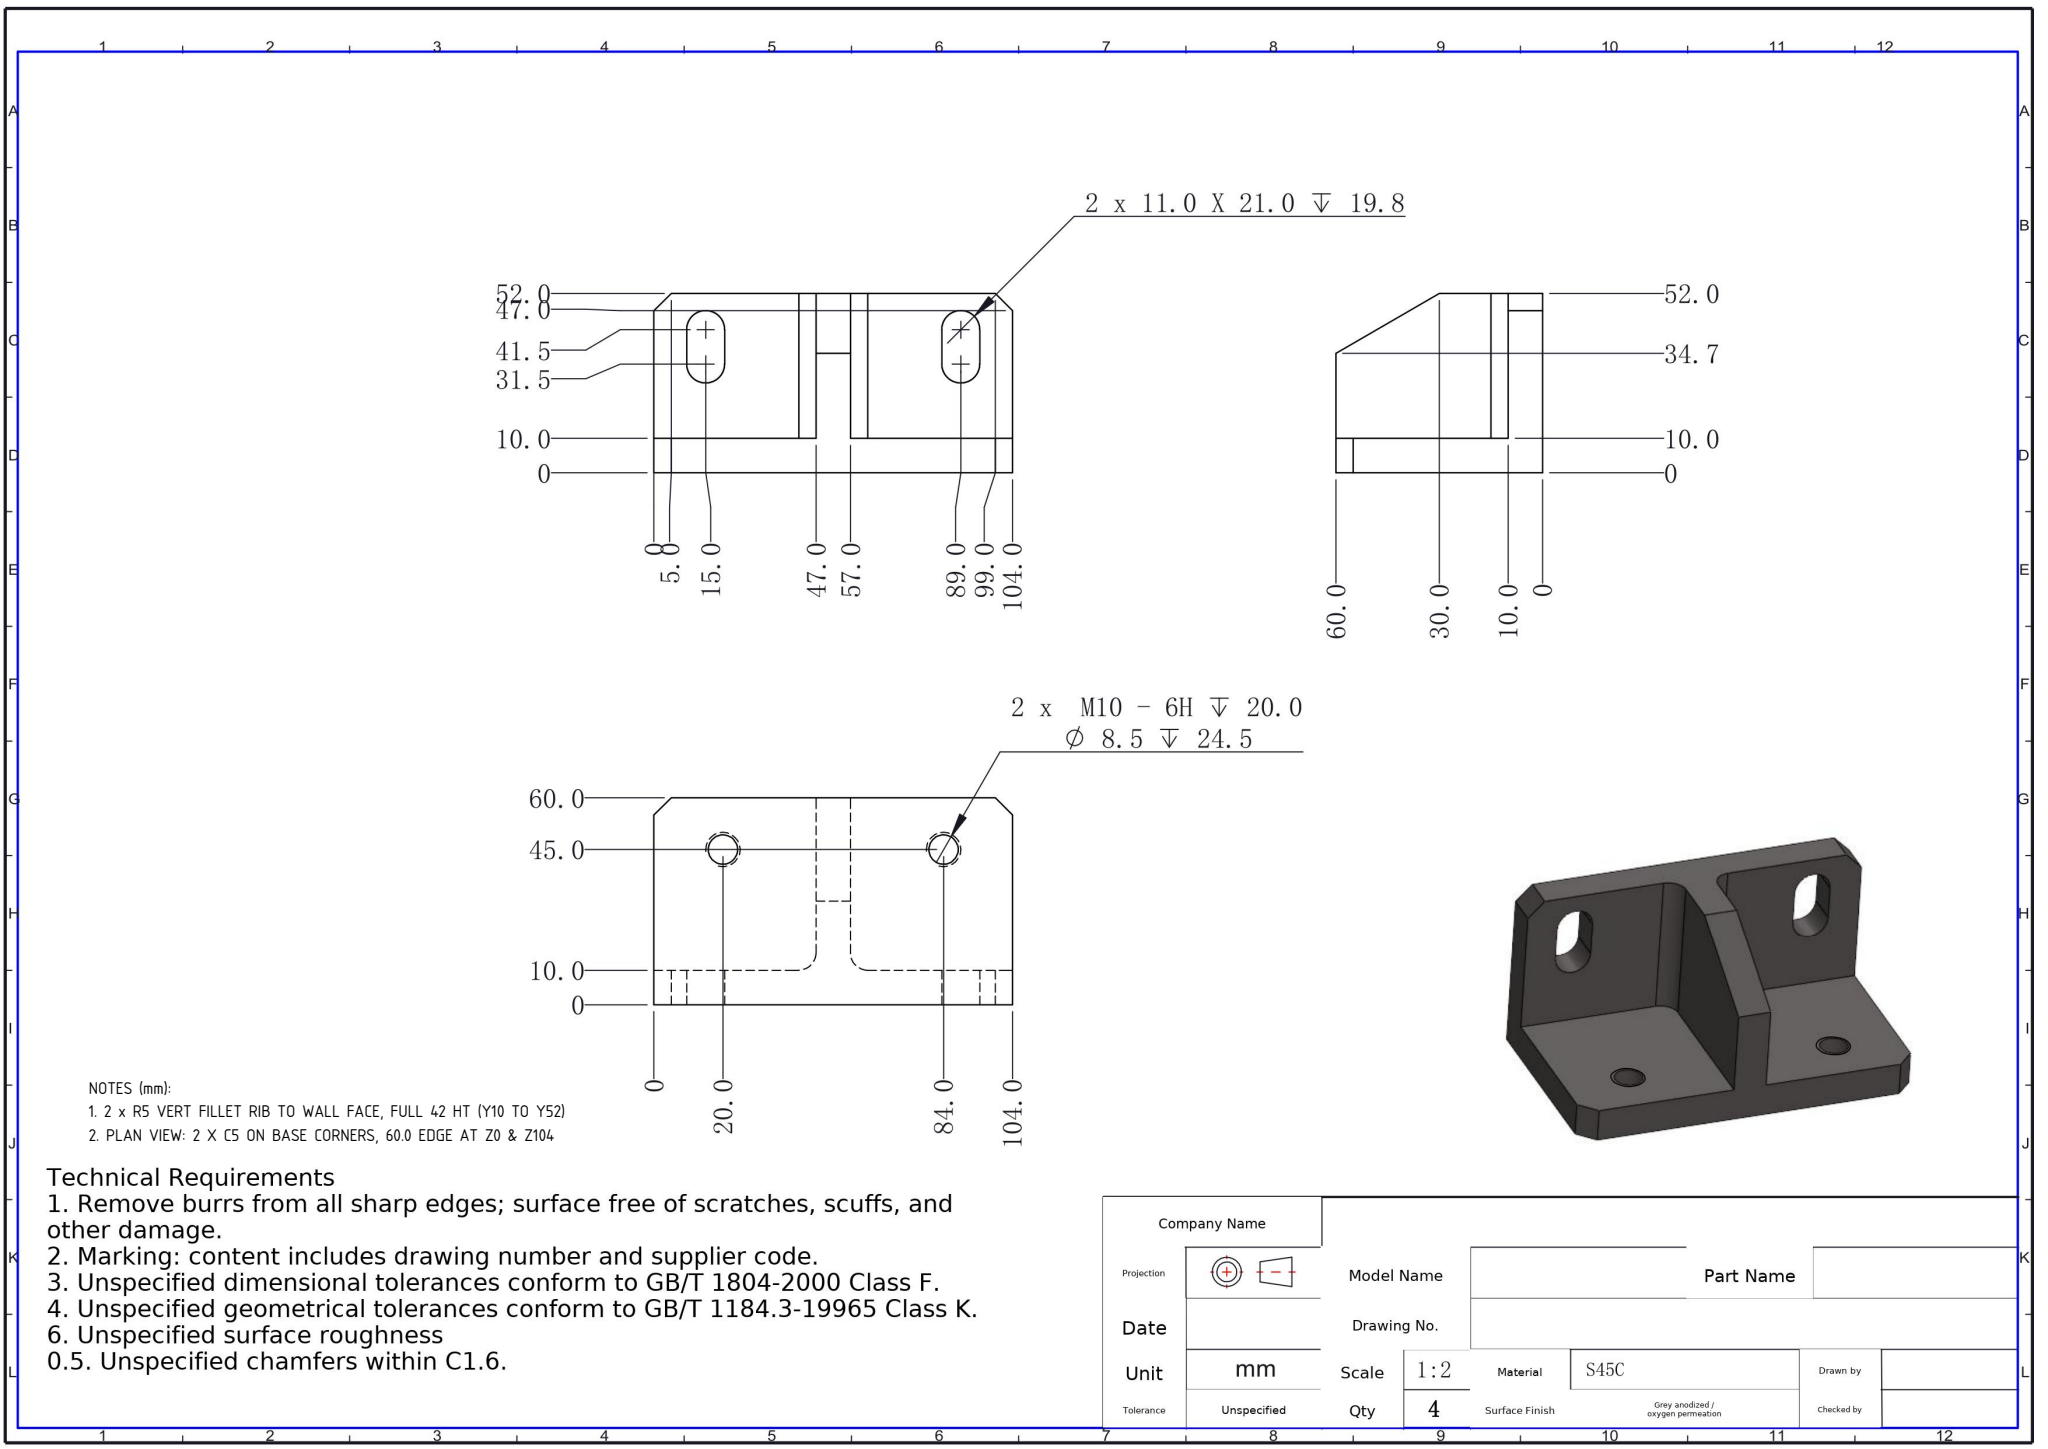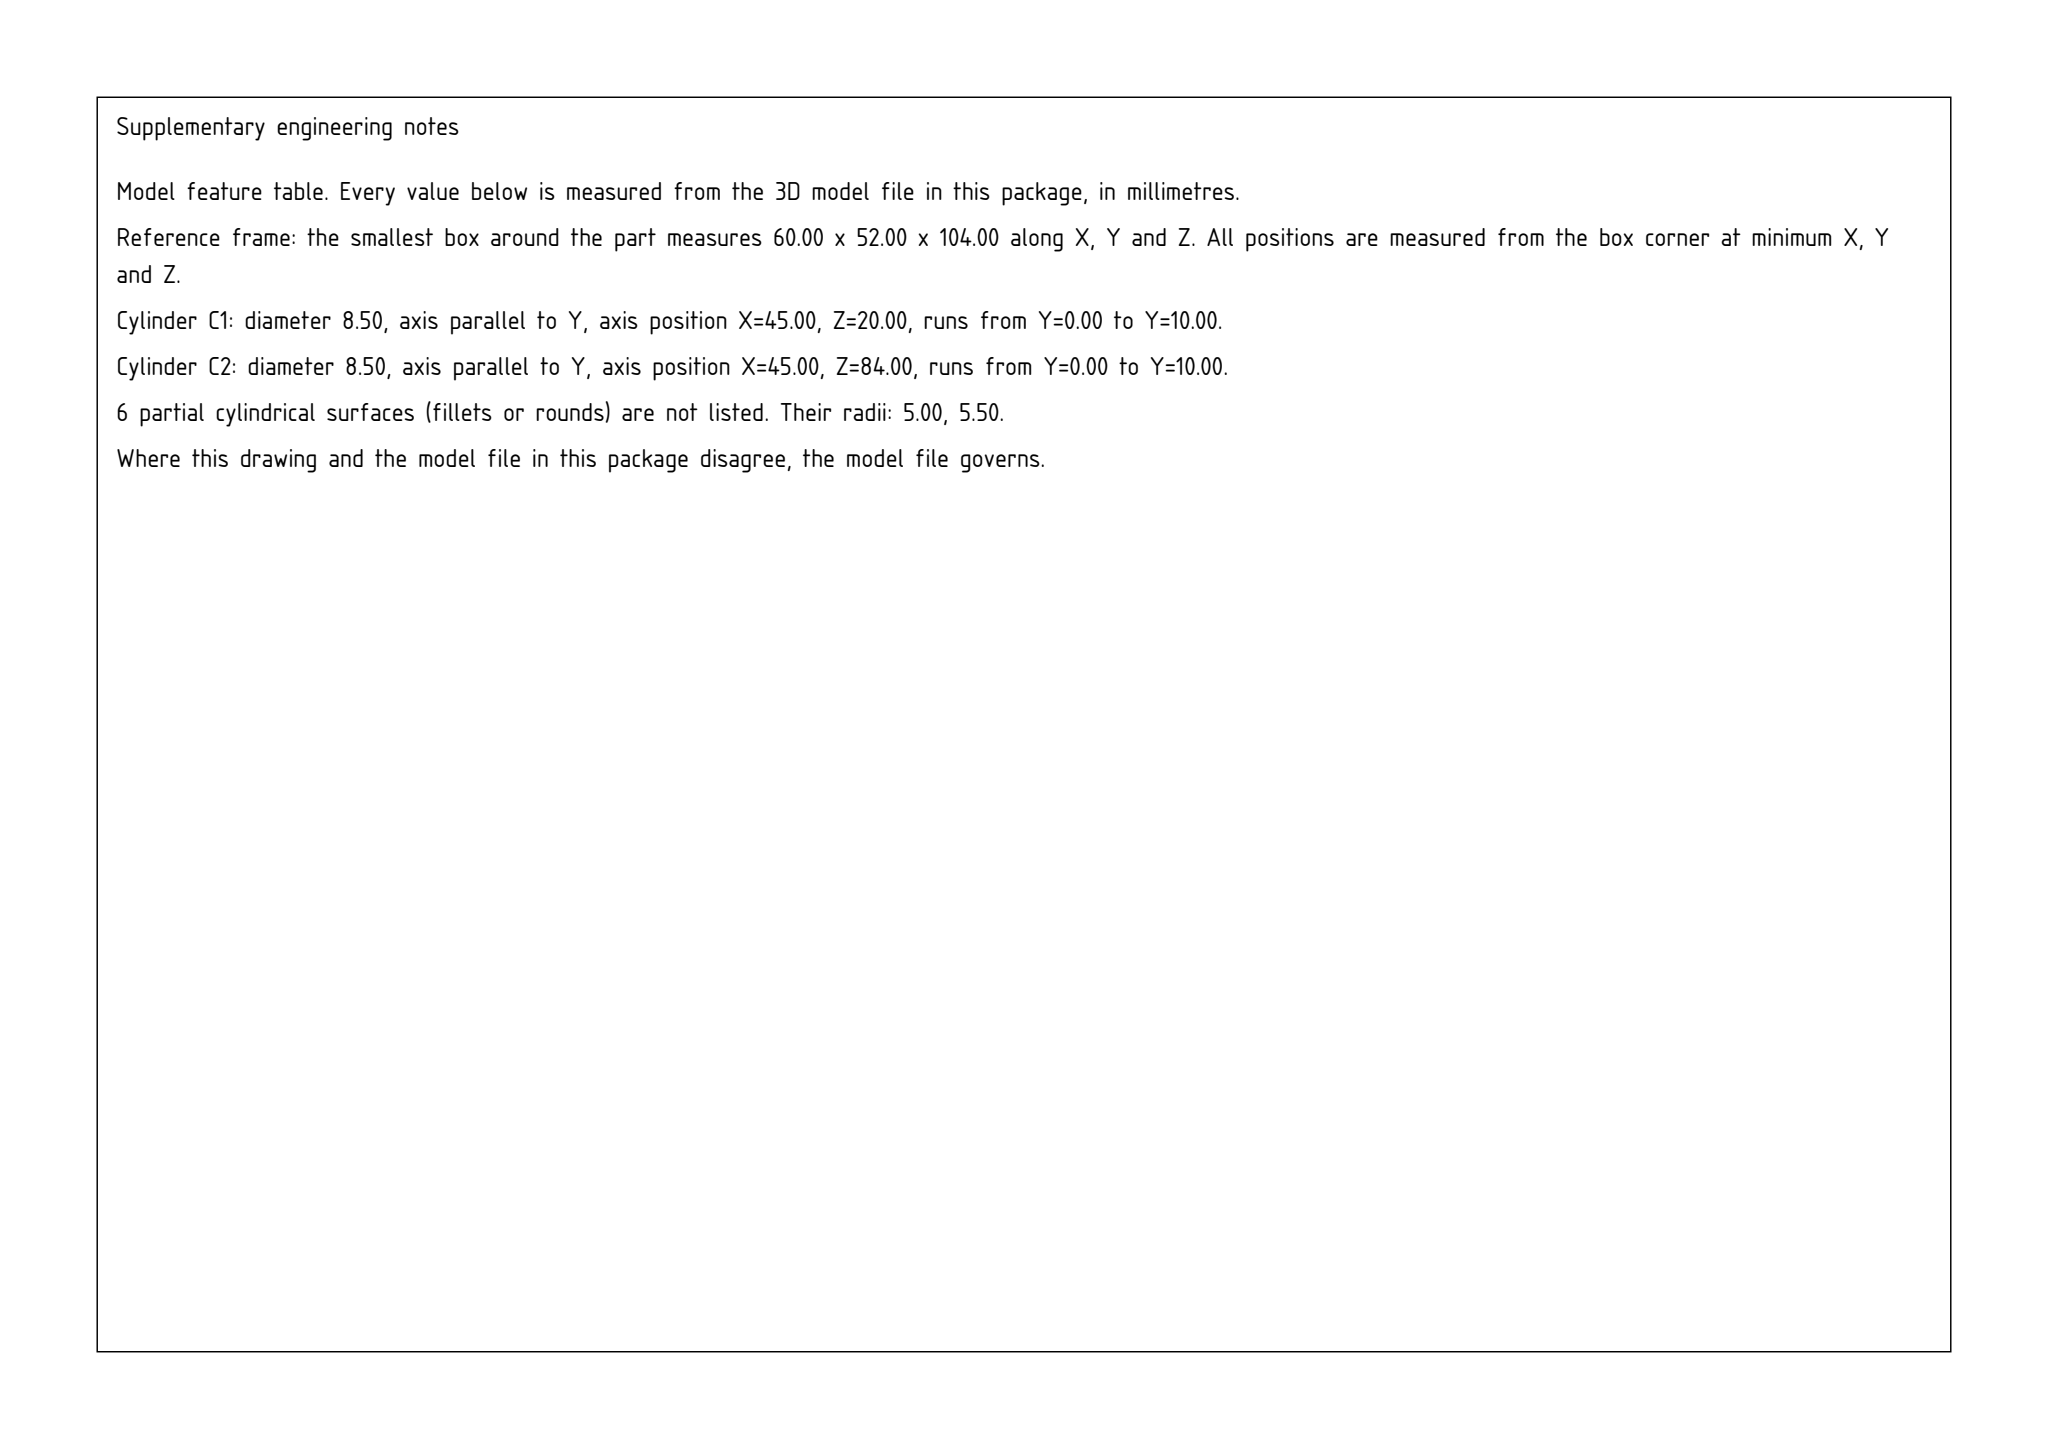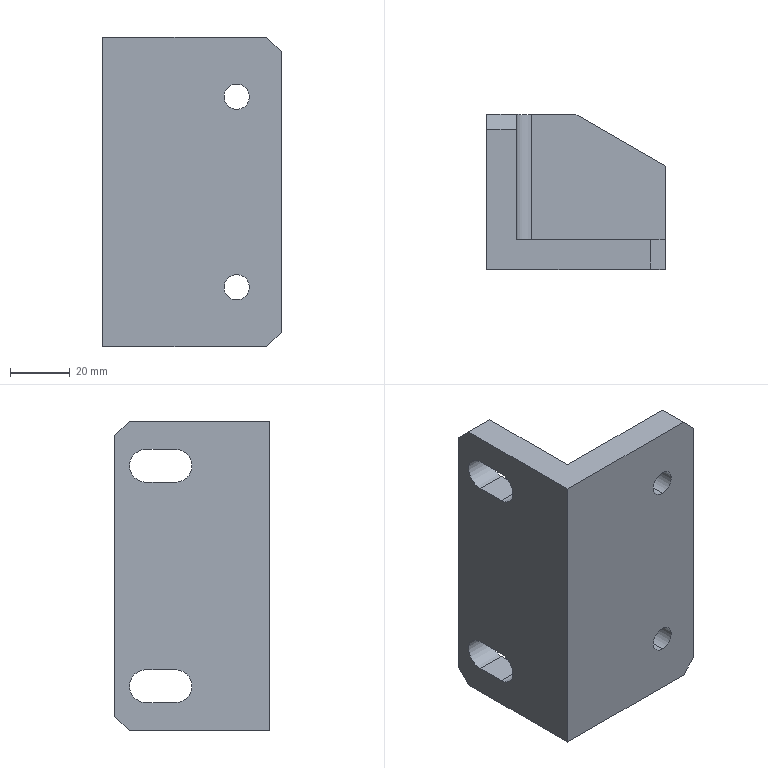Part | SolidWorks | mm | 1 solid | 31 faces | box 60 x 52 x 104 mm | volume 119197 mm3 | plane 21 | cylinder 10 | commonest cylinder face diameters 8.5 x4 11 x4 10 x2
Drawing notes:
2 x R5 VERT FILLET RIB TO WALL FACE, FULL 42 HT (Y10 TO Y52) | from the solid: cylinders dia 10, axis y, pos (x=15, z=42) and (x=15, z=62), length 42; wall face plane x=10, rib faces z=47 & z=57 -> R5 tangent blends
PLAN VIEW: 2 X C5 ON BASE CORNERS, 60.0 EDGE AT Z0 & Z104 | from the solid: Base plate bbox 60 (x) x 104 (z), y0-10; outer edge face x=60 and end faces z=0/z=104 meet at corners cut by two 45 deg planar faces (non axis-aligned, so absent from axis_planes list); cut extent 5 x 5 taken from corner of x=60/z=0 and x=60/z=104